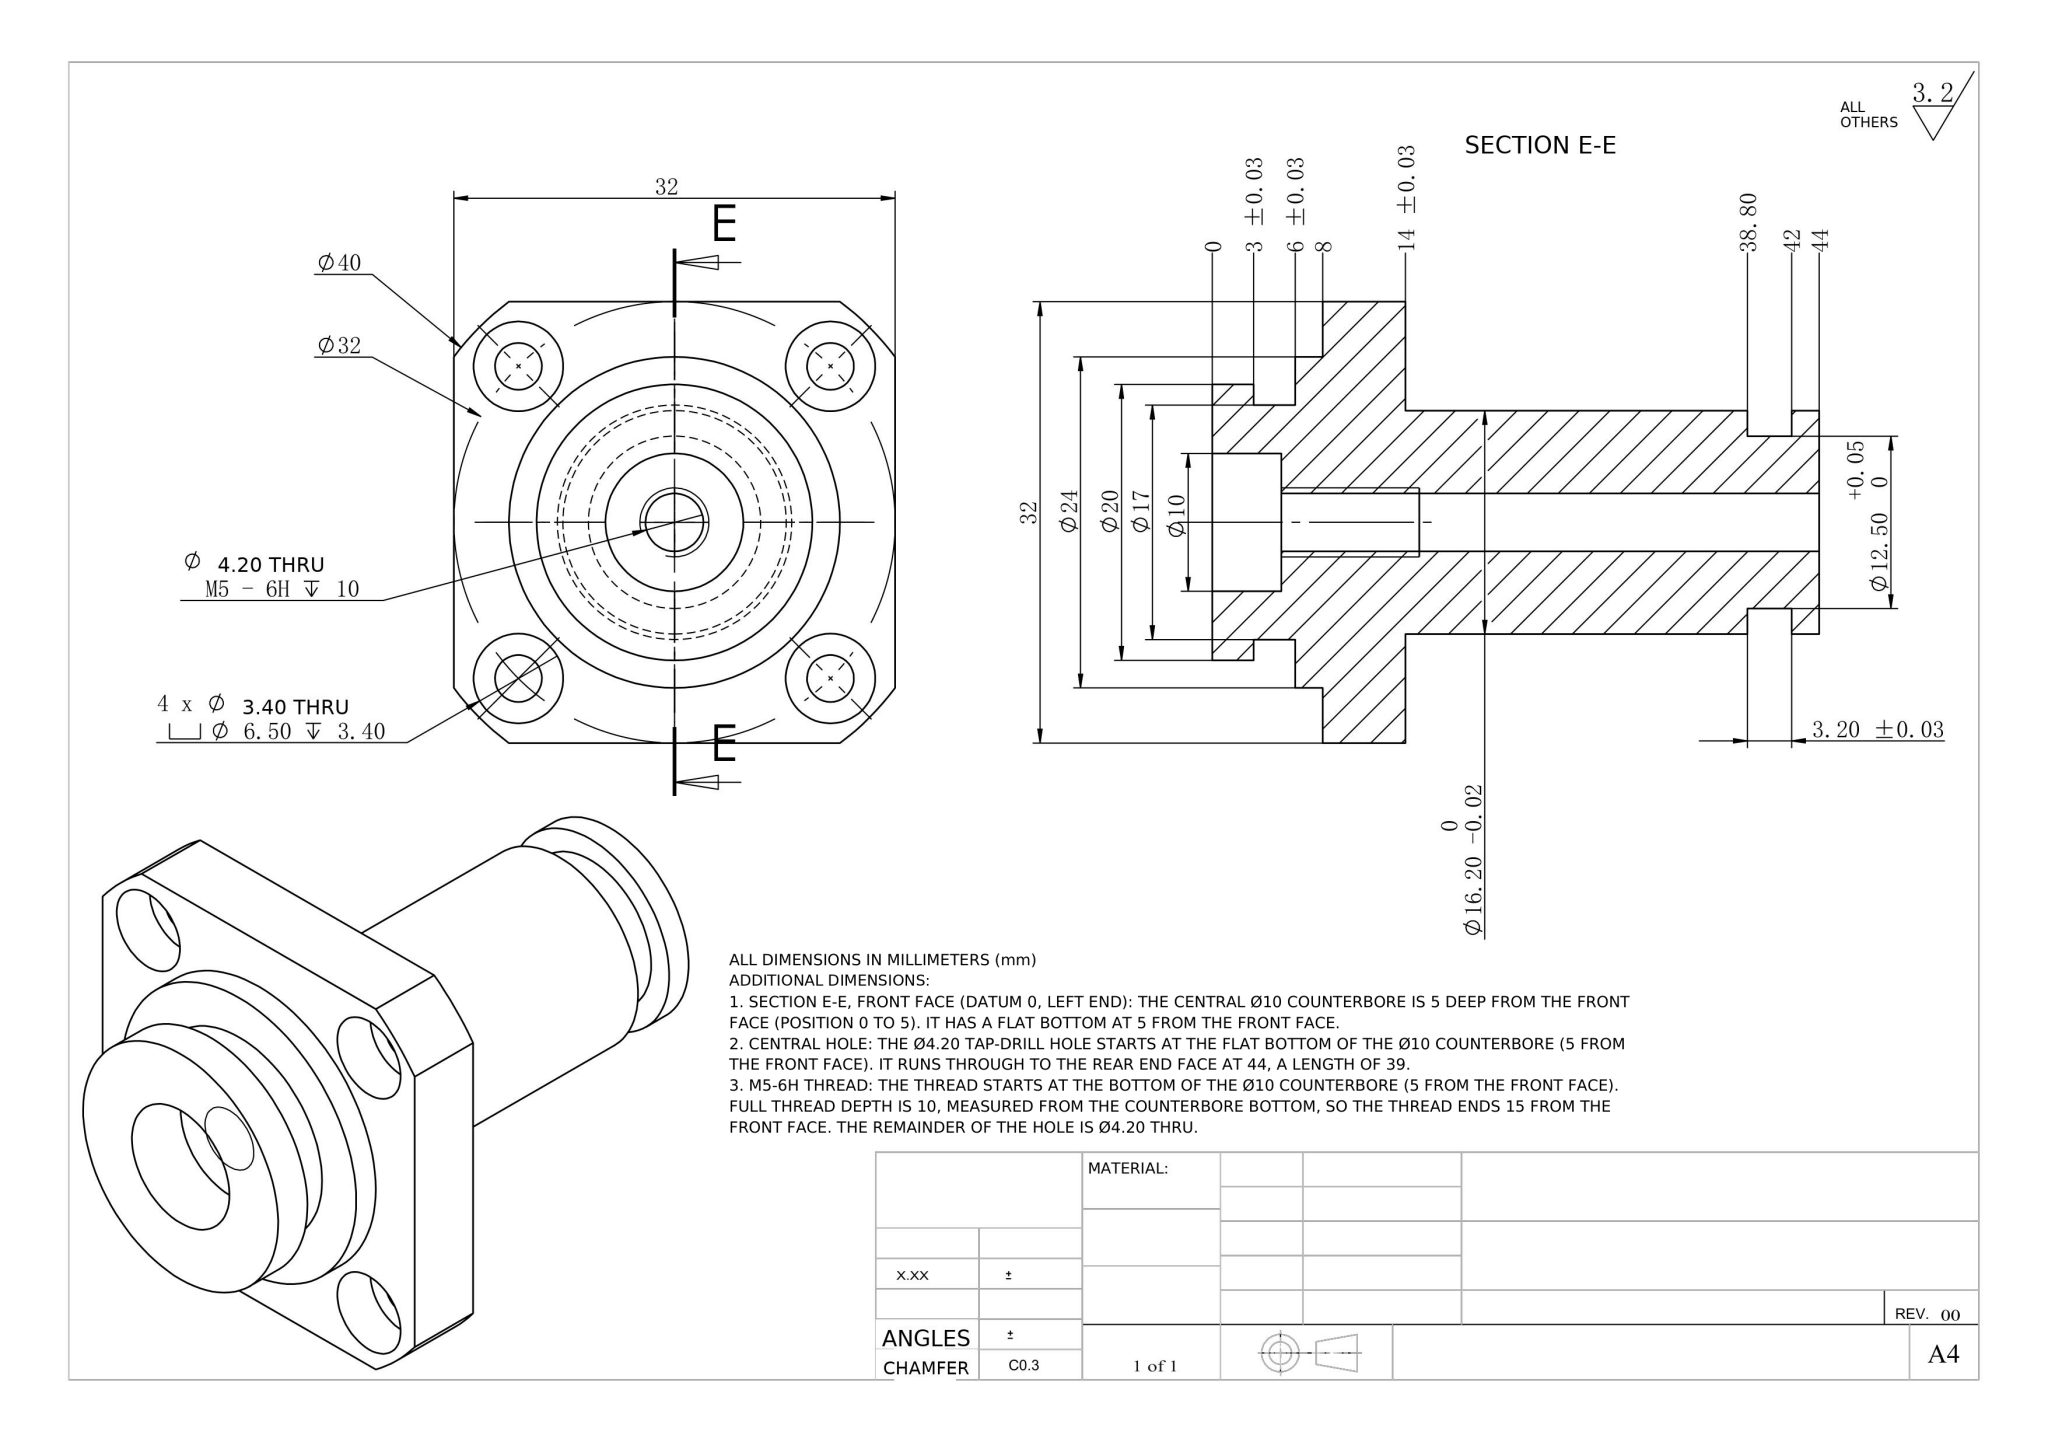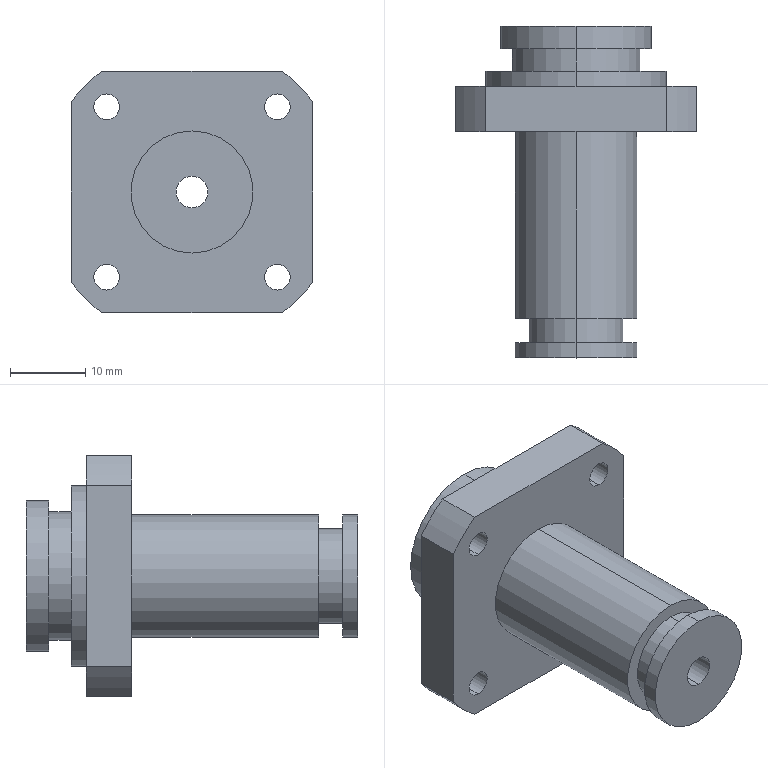Part | NX | mm | Square Flanged Stub Shaft | 1 solid | 53 faces | box 32 x 44 x 32 mm | volume 12936 mm3 | cylinder 36 | plane 17 | commonest cylinder face diameters 6.5 x8 3.4 x8 16.2 x4 40 x4 12.5 x2 4.2 x2 10 x2 20 x2